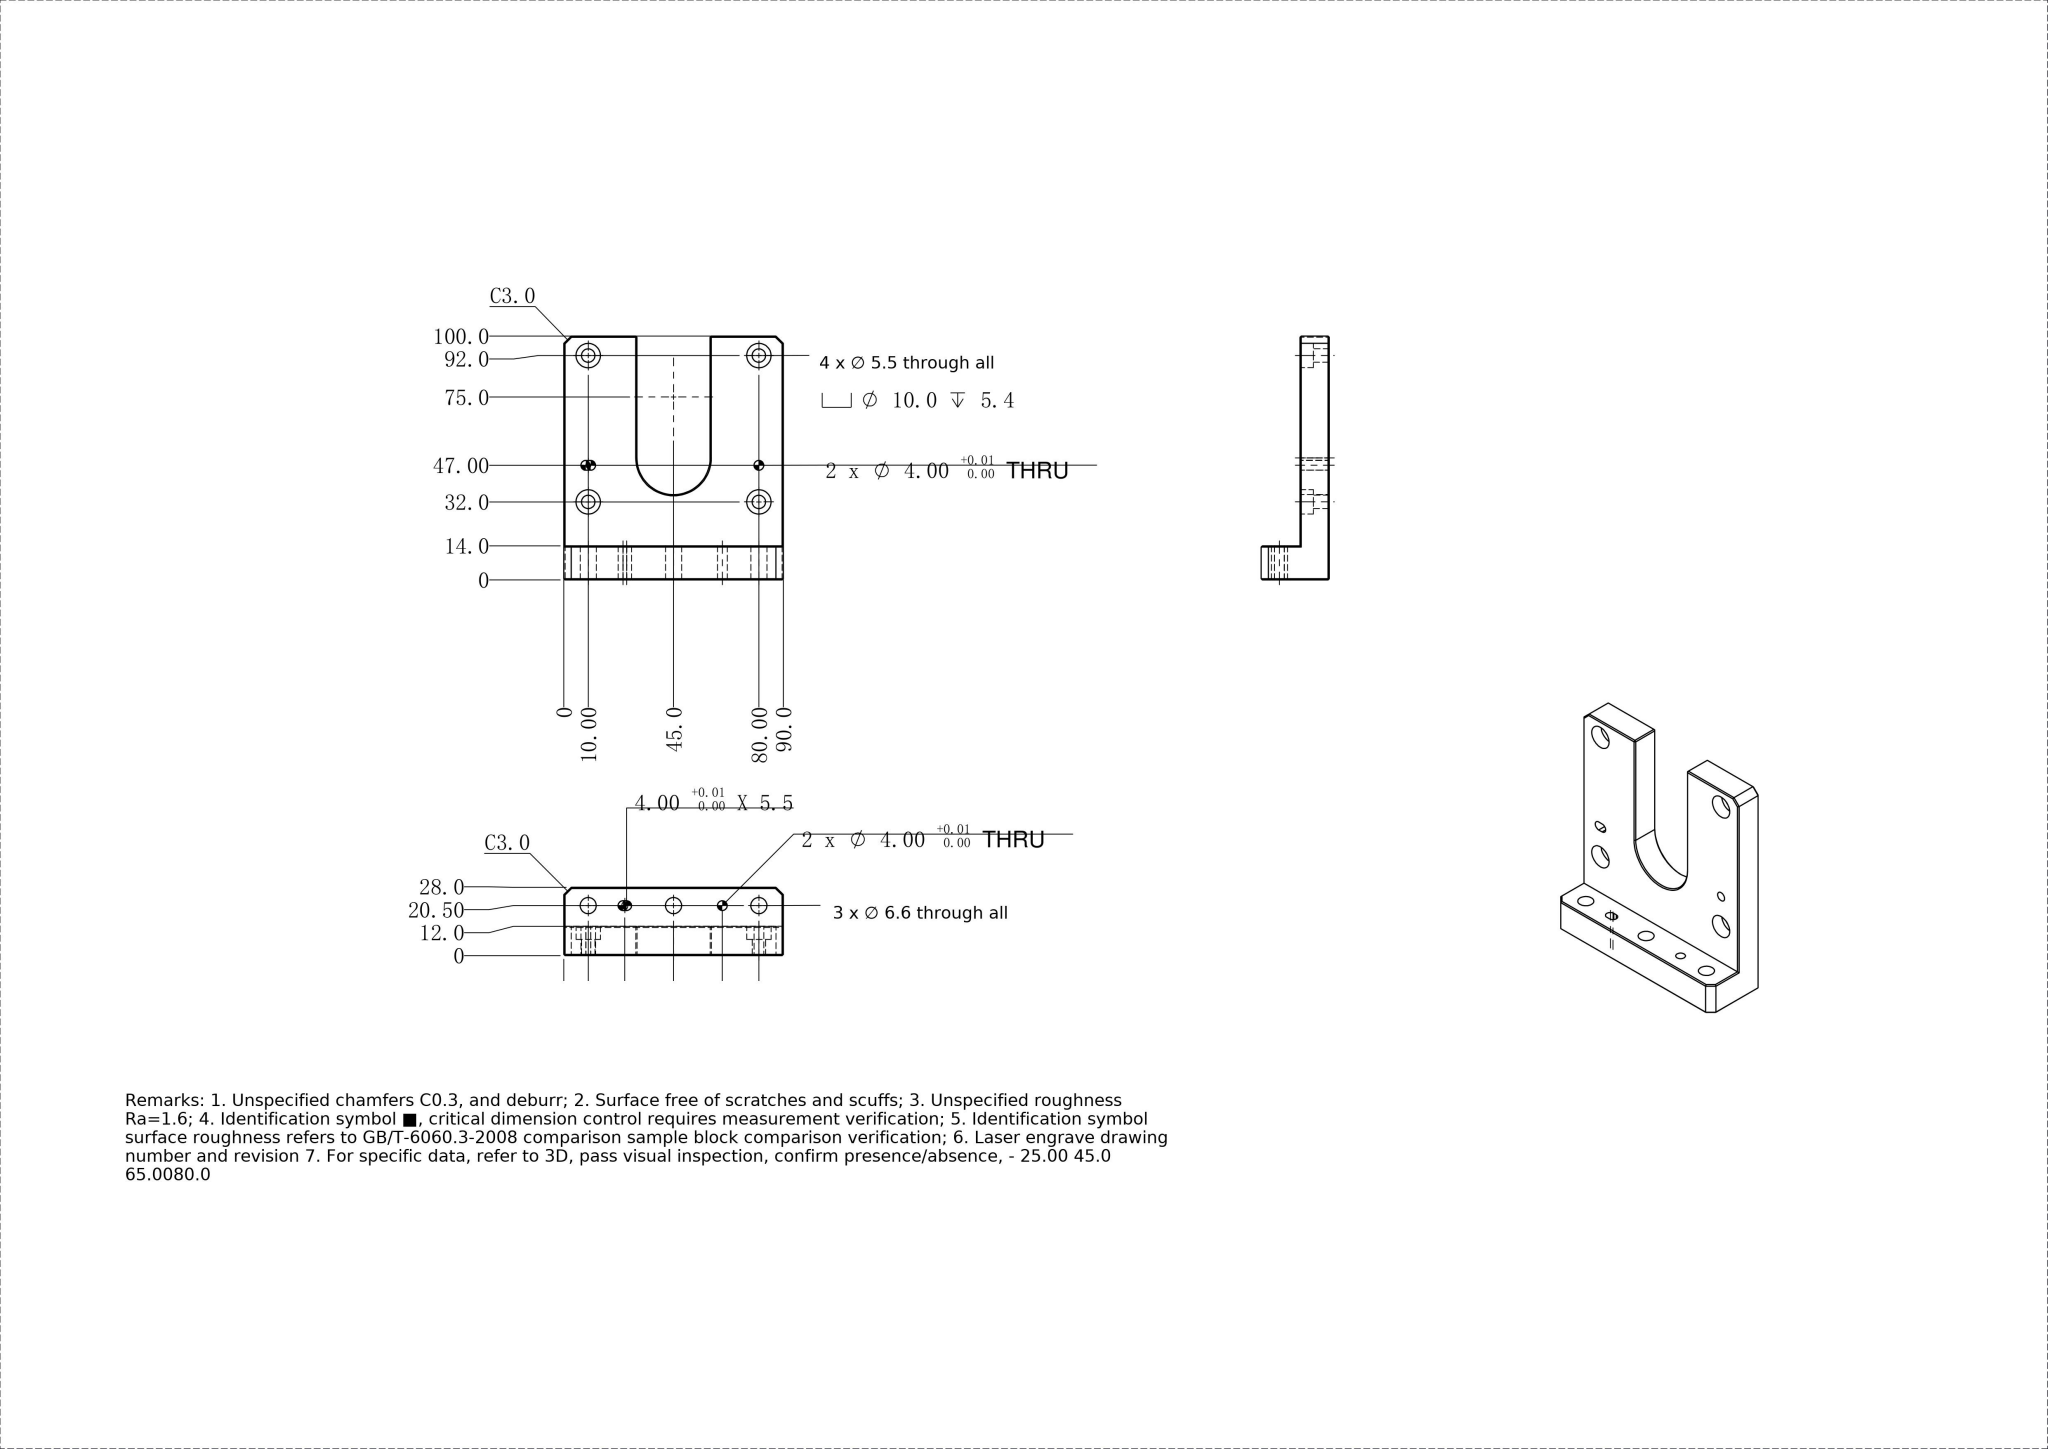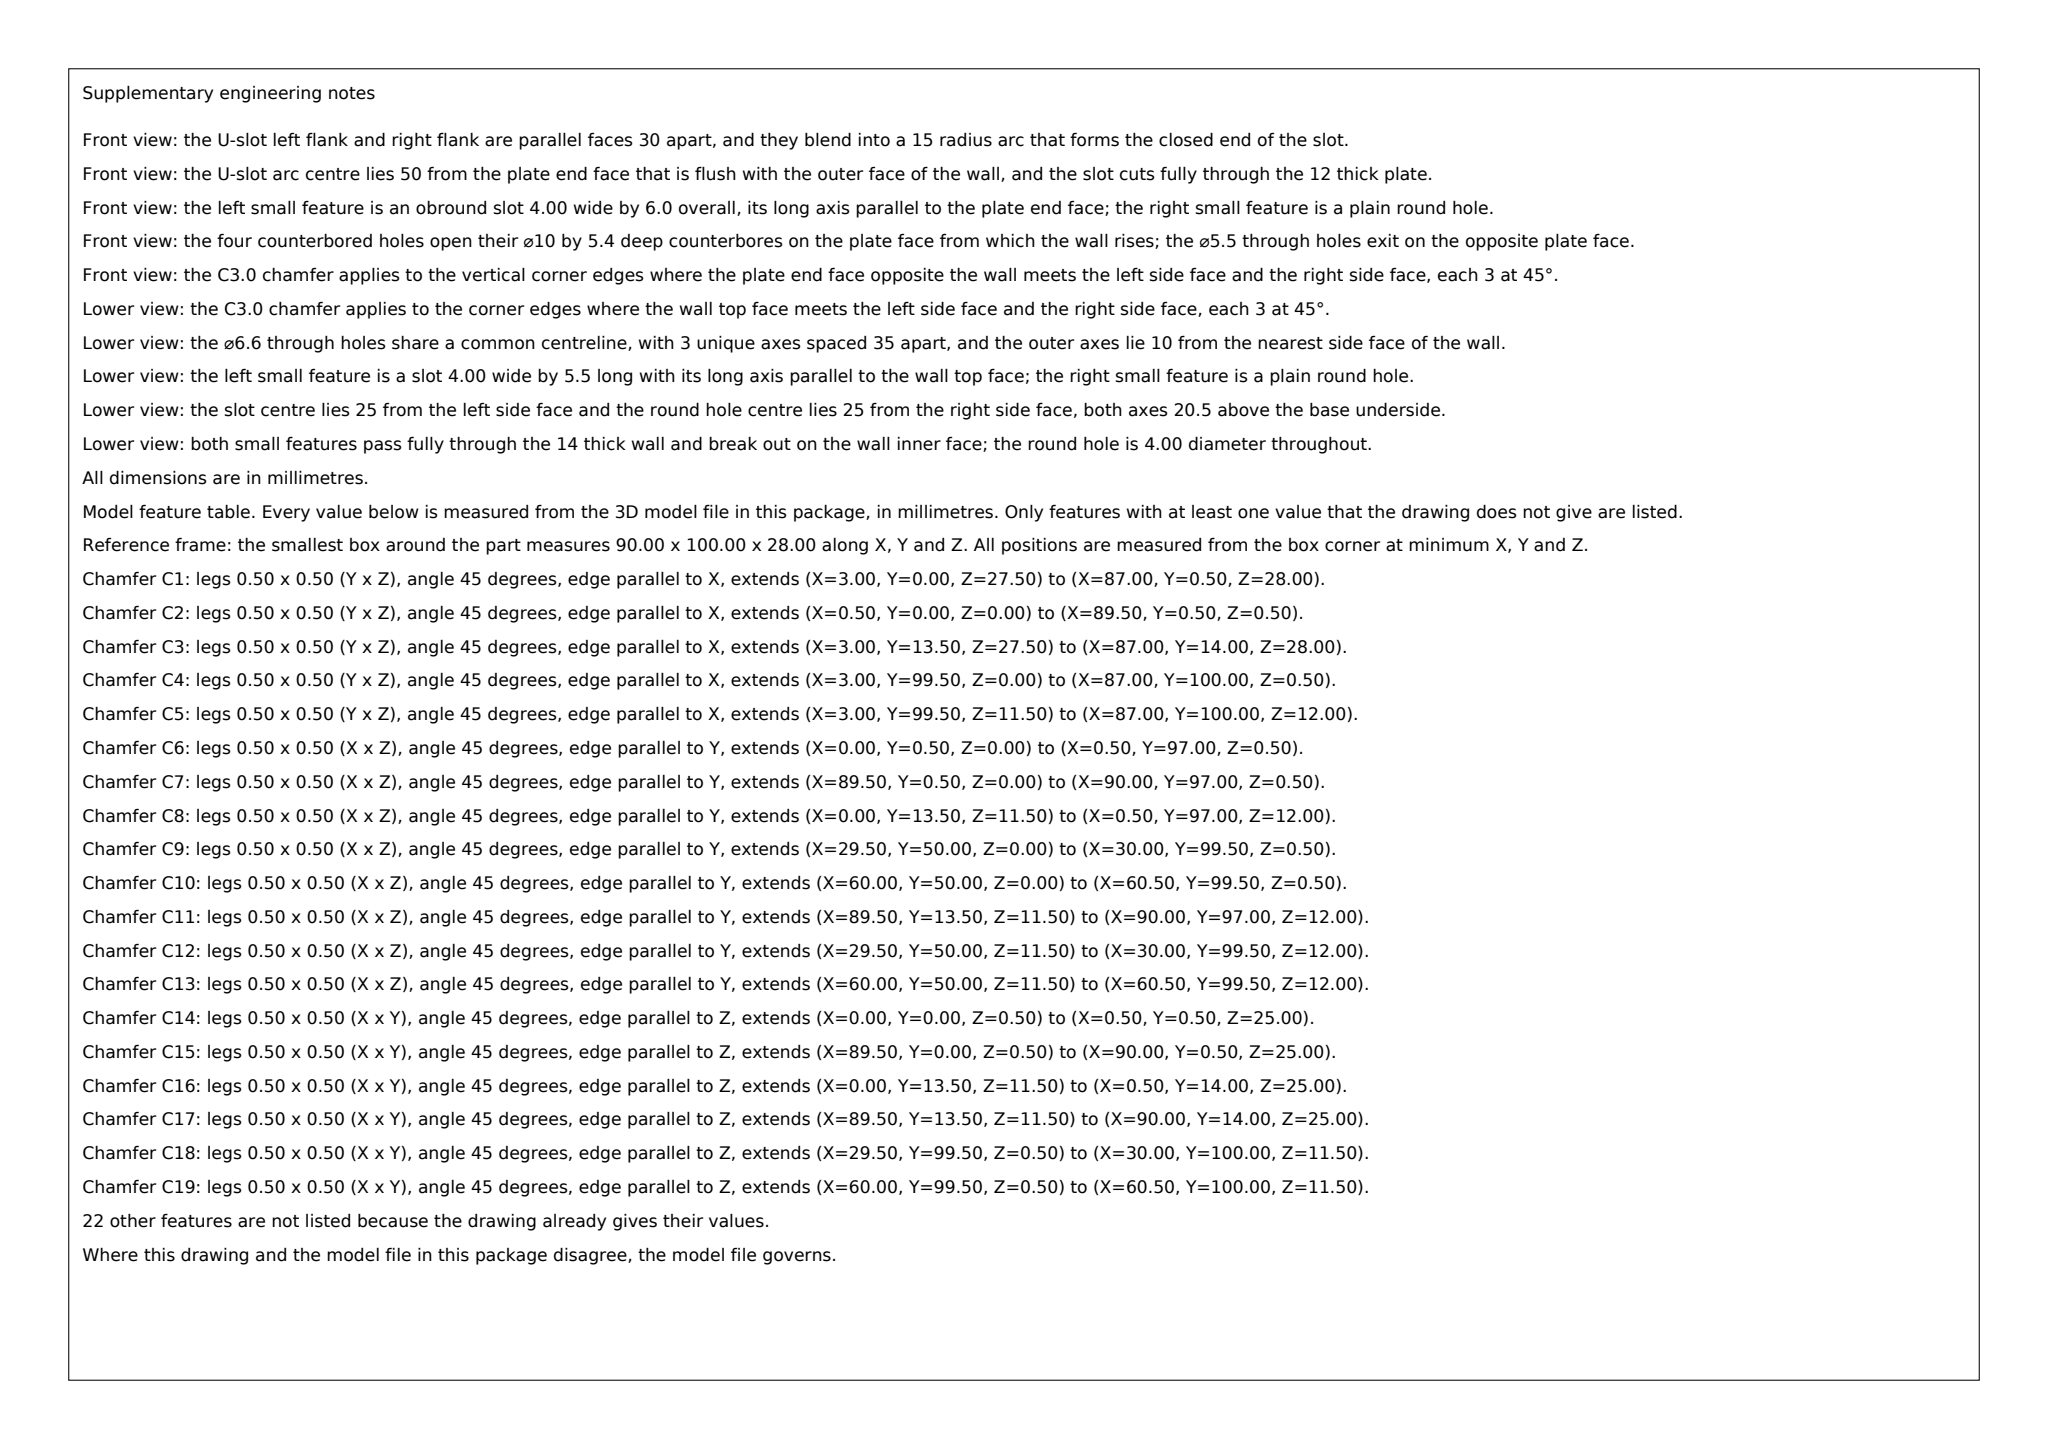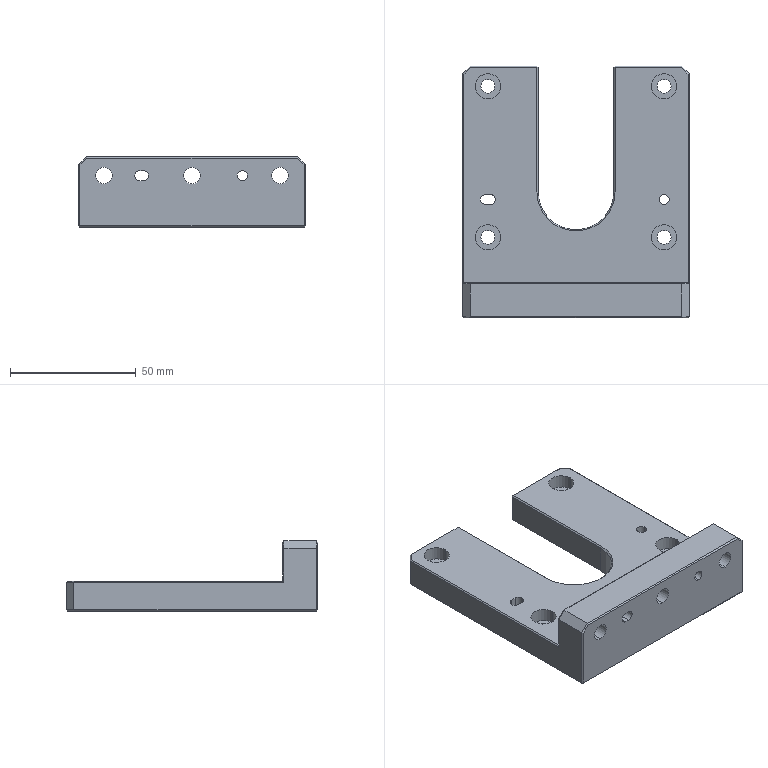Part | SolidWorks | mm | 1 solid | 92 faces | box 90 x 100 x 28 mm | volume 100947 mm3 | plane 58 | cylinder 32 | cone 2 | commonest cylinder face diameters 4 x9 10 x8 5.5 x8 6.6 x6 30 x1
Drawing notes:
U-SLOT 30.0 WIDE x R15.0 BOT, CL 45.0 FROM LH EDGE, R CTR 50.0 ABOVE BASE | from the solid: cyl dia 30.0 axis z at x=45.0, y=50.0, open to y=100 top face
SLOT 4.00 (+0.01/0) WIDE X 5.5 LG THRU (14.0), CL 25.0 FROM LH EDGE, 20.5 ABOVE BASE | from the solid: cylinders dia 4.0 axis y at (x=24.25, z=20.5) and (x=25.75, z=20.5), length 14.0
Ø4.00 (+0.01/0) THRU (14.0), 65.0 FROM LH EDGE, 20.5 ABOVE BASE | from the solid: cylinder dia 4.0 axis y at (x=65.0, z=20.5), length 14.0
SLOT 4.00 WIDE X 6.0 LG, DEPTH 12.0 FROM TOP FACE, CL 10.0 FROM LH EDGE, 47.0 ABOVE BASE | from the solid: cylinders dia 4.0 axis z at (9.0,47.0) and (11.0,47.0), length 12.0
3X Ø6.6 THRU (14.0) IN BASE, 20.5 ABOVE BASE, AT 10.0, 45.0 AND 80.0 FROM LH EDGE | from the solid: cylinders dia 6.6 axis y at x=10.0, 45.0, 80.0, z=20.5, length 14.0
2X Ø4.00 (+0.01/0) DEEP 12.0 FROM TOP FACE, 47.0 ABOVE BASE, AT 80.0 FROM LH EDGE | from the solid: cylinder dia 4.0 axis z at (80.0,47.0), length 12.0
UPRIGHT PLATE: SLOT 4.00 WIDE x 6.0 LONG THRU 12.0 PLATE, SLOT CL AT X=10.0 FROM LH EDGE, Y=47.0 ABOVE BASE | from the solid: cylinders dia 4.0 axis z at (9.0,47.0) and (11.0,47.0), length 12.0
BASE: SLOT 4.00(+0.01/0) WIDE x 5.5 LONG THRU 14.0 BASE, SLOT CL AT X=25.0 FROM LH EDGE, Z=20.5 FROM REAR FACE | from the solid: cylinders dia 4.0 axis y at (x=24.25,z=20.5) and (x=25.75,z=20.5), length 14.0
BASE: 2 x Ø4.00(+0.01/0) THRU 14.0 BASE AT X=65.0 FROM LH EDGE, Z=20.5 FROM REAR FACE | from the solid: cylinders dia 4.0 axis y at (x=65.0,z=20.5), length 14.0, count 2
U-SLOT: Ø30.0 (R15.0) THRU 12.0 PLATE, SLOT CL AT X=45.0 FROM LH EDGE, ARC CTR 50.0 ABOVE BASE | from the solid: cylinders: concave arc dia 30.0, axis z at [45.0, 50.0], from z=0.5 to 11.5, 180 deg
U-SLOT Ø30 EDGES: C0.5 X 45° (Ø30 TO Ø31) ON BOTH FACES OF THE 12.0 THK UPRIGHT PLATE | from the solid: cones: 90° included, ref dia 30.0 at z=11.5 and ref dia 31.0 at z=0.0, bbox x 29.5-60.5, y 34.5-50.0
C3.0 CHAMFER 2X ON UPRIGHT PLATE VERTICAL CORNERS AT X=0 AND X=90.0 FROM LH EDGE, Y=100.0 (TOP EDGE), FULL 12.0 PLATE THICKNESS | from the solid: inclined_planes 45/45/90 at bbox_from [0.0,97.0,0.5] and [87.0,97.0,0.5], size [3.0,3.0,11.0]
C3.0 CHAMFER 2X ON BASE TOP CORNERS AT X=0 AND X=90.0 FROM LH EDGE, ALONG TOP FACE Z=28.0, 14.0 LONG (FULL BASE DEPTH) | from the solid: inclined_planes 45/90/45 at bbox_from [0.0,0.5,25.0] and [87.0,0.5,25.0], size [3.0,13.0,3.0]
build123d program:
from build123d import *

# Parameters (mm, degrees)
SKETCH1_W                                       = 90
SKETCH1_H                                       = 100
BOSS_EXTRUDE1_DEPTH                             = 12
SKETCH2_W                                       = 90
SKETCH2_H                                       = 14
BOSS_EXTRUDE2_DEPTH                             = 16
CHAMFER1_SIZE                                   = 3
CUT_EXTRUDE1_DEPTH                              = 16
CHAMFER2_SIZE                                   = 0.5
M6_CLEARANCE_HOLE1_D                            = 6.6
M5_HEX_SOCKET_HEAD_CAP_SCREW_CBORE1_D           = 5.5
M5_HEX_SOCKET_HEAD_CAP_SCREW_CBORE1_CBORE_D     = 10
M5_HEX_SOCKET_HEAD_CAP_SCREW_CBORE1_CBORE_DEPTH = 5.4
SIZE_MM_DOWEL_PIN_HOLE1_D                       = 4
SIZE_MM_DOWEL_PIN_HOLE2_D                       = 4
CUT_EXTRUDE2_DEPTH                              = 102.02
CUT_EXTRUDE3_DEPTH                              = 70.145


with BuildPart() as part:
    # Sketch1 → Boss-Extrude1 (new body)
    with BuildSketch(Plane.XY):
        Rectangle(SKETCH1_W, SKETCH1_H)
    extrude(amount=BOSS_EXTRUDE1_DEPTH)

    # Sketch2 → Boss-Extrude2 (add)
    with BuildSketch(Plane.XY.offset(12)):
        with Locations((0, -43)):
            Rectangle(SKETCH2_W, SKETCH2_H)
    extrude(amount=BOSS_EXTRUDE2_DEPTH)

    # Chamfer1
    chamfer1_edges = [part.edges().sort_by_distance(p)[0] for p in [
        (-45, -43, 28),
        (45, -43, 28),
        (-45, 50, 6),
        (45, 50, 6),
    ]]
    chamfer(chamfer1_edges, length=CHAMFER1_SIZE)

    # Sketch3 → Cut-Extrude1 (cut)
    with BuildSketch(Plane.XY.offset(12)):
        with BuildLine():
            Line((15, 50), (15, 0))
            ThreePointArc((15, 0), (0, -15), (-15, 0))
            Line((-15, 0), (-15, 50))
            ThreePointArc((-15, 50), (0, 65), (15, 50))
        make_face()
    extrude(amount=-CUT_EXTRUDE1_DEPTH, mode=Mode.SUBTRACT)

    # Chamfer2
    chamfer2_edges = [part.edges().sort_by_distance(p)[0] for p in [
        (45, 5.5, 12),
        (0, -50, 28),
        (0, -36, 28),
        (-45, -36, 18.5),
        (45, -36, 18.5),
        (-43.5, -36, 26.5),
        (43.5, -36, 26.5),
        (45, -50, 12.5),
        (-45, -50, 12.5),
        (-43.5, -50, 26.5),
        (43.5, -50, 26.5),
        (-45, -1.5, 0),
        (-45, 5.5, 12),
        (28.5, 50, 0),
        (28.5, 50, 12),
        (-43.5, 48.5, 0),
        (43.5, 48.5, 0),
        (-43.5, 48.5, 12),
        (43.5, 48.5, 12),
        (0, -50, 0),
        (-28.5, 50, 0),
        (-15, 25, 0),
        (0, -15, 0),
        (15, 25, 0),
        (-28.5, 50, 12),
        (15, 25, 12),
        (-15, 25, 12),
        (0, -15, 12),
        (15, 50, 6),
        (-15, 50, 6),
        (45, -1.5, 0),
    ]]
    chamfer(chamfer2_edges, length=CHAMFER2_SIZE)

    # M6 Clearance Hole1 (through all)
    with Locations(Plane(origin=(0, -36, 0), x_dir=(1, 0, 0), z_dir=(0, 1, 0))):
        with Locations((-35, -20.5), (35, -20.5), (0, -20.5)):
            Hole(M6_CLEARANCE_HOLE1_D / 2)

    # M5 Hex Socket Head Cap Screw CBORE1 (through all)
    with Locations(Plane.XY.offset(12)):
        with Locations((-35, 42), (-35, -18), (35, 42), (35, -18)):
            CounterBoreHole(M5_HEX_SOCKET_HEAD_CAP_SCREW_CBORE1_D / 2, M5_HEX_SOCKET_HEAD_CAP_SCREW_CBORE1_CBORE_D / 2, M5_HEX_SOCKET_HEAD_CAP_SCREW_CBORE1_CBORE_DEPTH)

    # Size mm Dowel Pin Hole1 (through all)
    with Locations(Plane.XY.offset(12)):
        with Locations((-35, -3), (35, -3)):
            Hole(SIZE_MM_DOWEL_PIN_HOLE1_D / 2)

    # Size mm Dowel Pin Hole2 (through all)
    with Locations(Plane(origin=(0, -36, 0), x_dir=(1, 0, 0), z_dir=(0, 1, 0))):
        with Locations((-20, -20.5), (20, -20.5)):
            Hole(SIZE_MM_DOWEL_PIN_HOLE2_D / 2)

    # Sketch12 → Cut-Extrude2 (cut, through all)
    with BuildSketch(Plane(origin=(0, -36, 0), x_dir=(1, 0, 0), z_dir=(0, 1, 0))):
        with BuildLine():
            Line((-20.75, -18.5), (-19.25, -18.5))
            ThreePointArc((-19.25, -18.5), (-17.25, -20.5), (-19.25, -22.5))
            Line((-19.25, -22.5), (-20.75, -22.5))
            ThreePointArc((-20.75, -22.5), (-22.75, -20.5), (-20.75, -18.5))
        make_face()
    extrude(amount=-CUT_EXTRUDE2_DEPTH, mode=Mode.SUBTRACT)

    # Sketch13 → Cut-Extrude3 (cut, through all)
    with BuildSketch(Plane.XY.offset(12)):
        with BuildLine():
            Line((-36, -1), (-34, -1))
            ThreePointArc((-34, -1), (-32, -3), (-34, -5))
            Line((-34, -5), (-36, -5))
            ThreePointArc((-36, -5), (-38, -3), (-36, -1))
        make_face()
    extrude(amount=-CUT_EXTRUDE3_DEPTH, mode=Mode.SUBTRACT)


solid = part.part